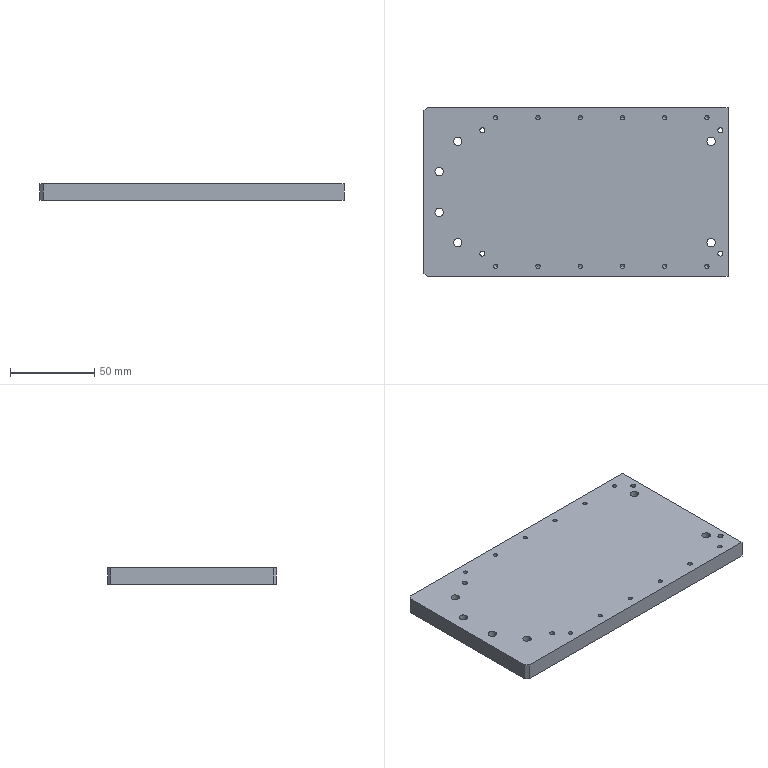Component | SolidWorks | 200-02-1 | 1 solid | 76 faces | box 180 x 100 x 10 mm | volume 178043 mm3 | cylinder 44 | cone 24 | plane 8 | commonest cylinder face diameters 2.5 x24 5 x12 3 x8 | material 6061
build123d program:
from build123d import *

# Parameters (mm, degrees)
SKETCH1_W                 = 180
SKETCH1_H                 = 100
BOSS_EXTRUDE1_DEPTH       = 5
LPATTERN1_COUNT           = 6
LPATTERN1_PITCH           = 25
SIZE_MM_DOWEL_PIN_HOLE1_D = 3
M6_TAPPED_HOLE3_D         = 5
CHAMFER1_SIZE             = 2
M6_TAPPED_HOLE2_D         = 5


with BuildPart() as part:
    # Sketch1 → Boss-Extrude1 (new, symmetric)
    with BuildSketch(Plane.XY):
        Rectangle(SKETCH1_W, SKETCH1_H)
    extrude(amount=BOSS_EXTRUDE1_DEPTH, both=True)

    # Sketch3 → M3 Tapped Hole1 (revolve, cut)
    with BuildSketch(Plane(origin=(77.5, 44, 5), x_dir=(0, -1, 0), z_dir=(1, 0, 0))):
        Polygon((0, 0), (0, 8.251), (1.25, 7.5), (1.25, 0), align=None)
    m3_tapped_hole1 = revolve(axis=Axis((77.5, 44, 11.35), (0, 0, -1)), mode=Mode.SUBTRACT)

    # LPattern1: M3 Tapped Hole1 ×6
    with Locations(*[(-i * LPATTERN1_PITCH, 0, 0) for i in range(1, LPATTERN1_COUNT)]):
        add(m3_tapped_hole1, mode=Mode.SUBTRACT)

    # Size mm Dowel Pin Hole1 (through all)
    with Locations(Plane.XY.offset(5)):
        with Locations((85.5, 36.5), (-55.5, 36.5)):
            size_mm_dowel_pin_hole1 = Hole(SIZE_MM_DOWEL_PIN_HOLE1_D / 2)

    # Mirror1: M3 Tapped Hole1, Size mm Dowel Pin Hole1 across plane
    add(m3_tapped_hole1.mirror(Plane.ZX), mode=Mode.SUBTRACT)
    add(size_mm_dowel_pin_hole1.mirror(Plane.ZX), mode=Mode.SUBTRACT)

    # Mirror1 copy 1 sketch → Mirror1 copy 1 (revolve, cut)
    with BuildSketch(Plane(origin=(52.5, -44, 5), x_dir=(0, 1, 0), z_dir=(1, 0, 0))):
        Polygon((0, 0), (0, -8.251), (1.25, -7.5), (1.25, 0), align=None)
    revolve(axis=Axis((52.5, -44, 11.35), (0, 0, 1)), mode=Mode.SUBTRACT)

    # Mirror1 copy 2 sketch → Mirror1 copy 2 (revolve, cut)
    with BuildSketch(Plane(origin=(27.5, -44, 5), x_dir=(0, 1, 0), z_dir=(1, 0, 0))):
        Polygon((0, 0), (0, -8.251), (1.25, -7.5), (1.25, 0), align=None)
    revolve(axis=Axis((27.5, -44, 11.35), (0, 0, 1)), mode=Mode.SUBTRACT)

    # Mirror1 copy 3 sketch → Mirror1 copy 3 (revolve, cut)
    with BuildSketch(Plane(origin=(2.5, -44, 5), x_dir=(0, 1, 0), z_dir=(1, 0, 0))):
        Polygon((0, 0), (0, -8.251), (1.25, -7.5), (1.25, 0), align=None)
    revolve(axis=Axis((2.5, -44, 11.35), (0, 0, 1)), mode=Mode.SUBTRACT)

    # Mirror1 copy 4 sketch → Mirror1 copy 4 (revolve, cut)
    with BuildSketch(Plane(origin=(-22.5, -44, 5), x_dir=(0, 1, 0), z_dir=(1, 0, 0))):
        Polygon((0, 0), (0, -8.251), (1.25, -7.5), (1.25, 0), align=None)
    revolve(axis=Axis((-22.5, -44, 11.35), (0, 0, 1)), mode=Mode.SUBTRACT)

    # Mirror1 copy 5 sketch → Mirror1 copy 5 (revolve, cut)
    with BuildSketch(Plane(origin=(-47.5, -44, 5), x_dir=(0, 1, 0), z_dir=(1, 0, 0))):
        Polygon((0, 0), (0, -8.251), (1.25, -7.5), (1.25, 0), align=None)
    revolve(axis=Axis((-47.5, -44, 11.35), (0, 0, 1)), mode=Mode.SUBTRACT)

    # M6 Tapped Hole3 (through all)
    with Locations(Plane.XY.offset(5)):
        with Locations((-81, 12)):
            m6_tapped_hole3 = Hole(M6_TAPPED_HOLE3_D / 2)

    # Mirror2: M6 Tapped Hole3 across plane
    add(m6_tapped_hole3.mirror(Plane.ZX), mode=Mode.SUBTRACT)

    # Chamfer1
    chamfer1_edges = [part.edges().sort_by_distance(p)[0] for p in [
        (-90, -50, 0),
        (-90, 50, 0),
    ]]
    chamfer(chamfer1_edges, length=CHAMFER1_SIZE)

    # M6 Tapped Hole2 (through all)
    with Locations(Plane(origin=(0, 0, -5), x_dir=(-1, 0, 0), z_dir=(0, 0, -1))):
        with Locations((-80, -30), (70, -30)):
            m6_tapped_hole2 = Hole(M6_TAPPED_HOLE2_D / 2)

    # Mirror3: M6 Tapped Hole2 across plane
    add(m6_tapped_hole2.mirror(Plane.ZX), mode=Mode.SUBTRACT)


solid = part.part

# Placed as in the assembly
solid = solid.moved(Location((190, 68, -80), (0, 0, 0)))